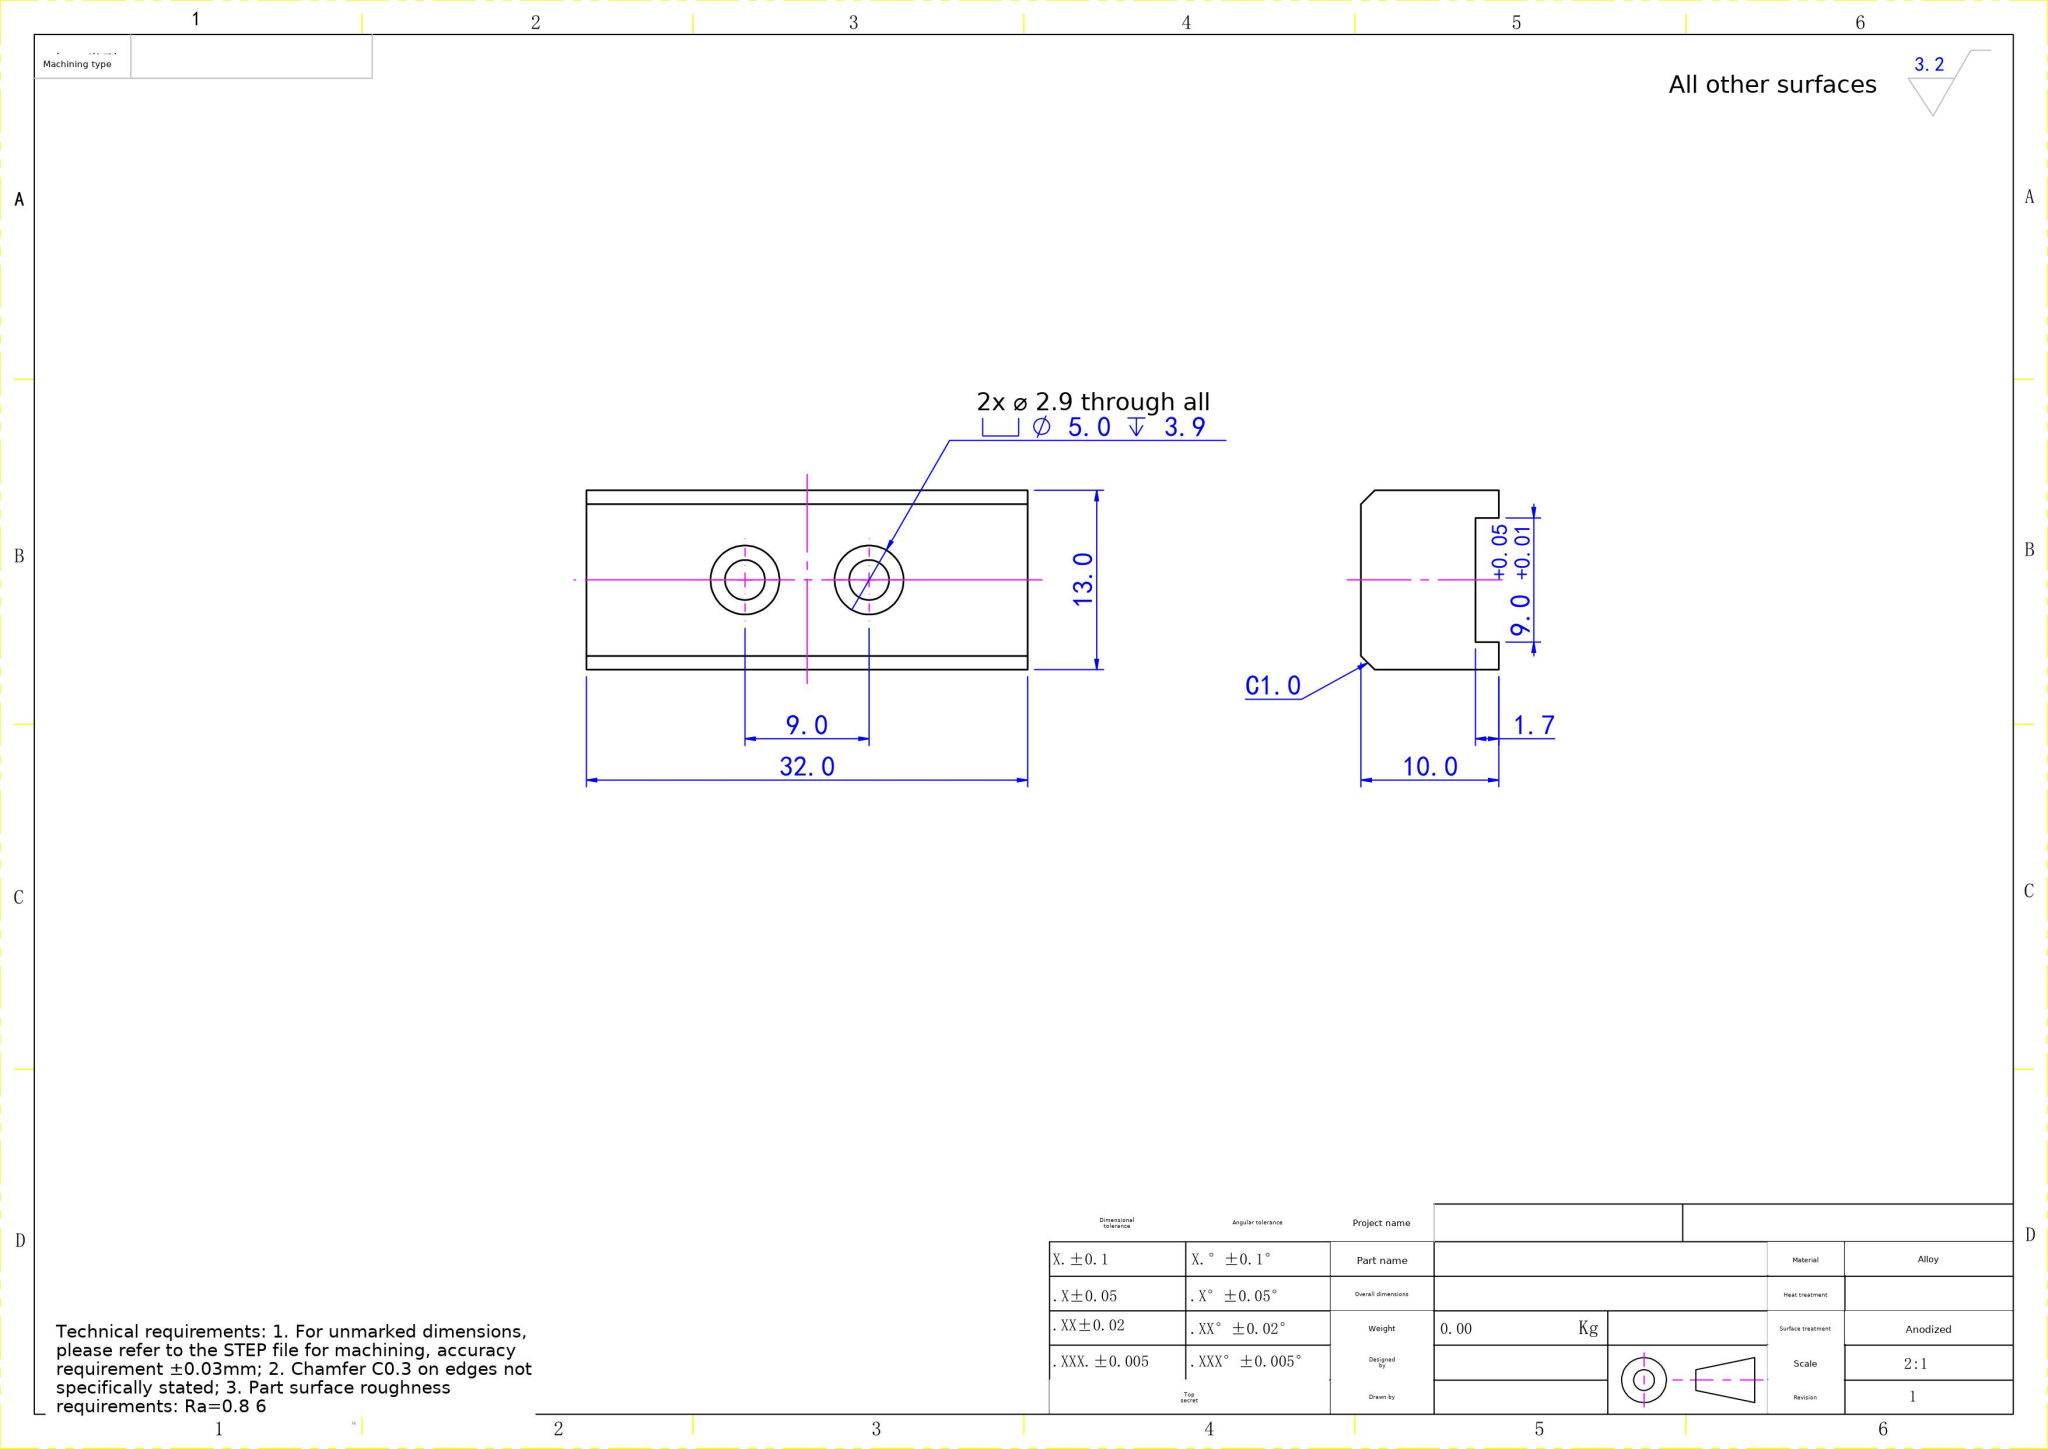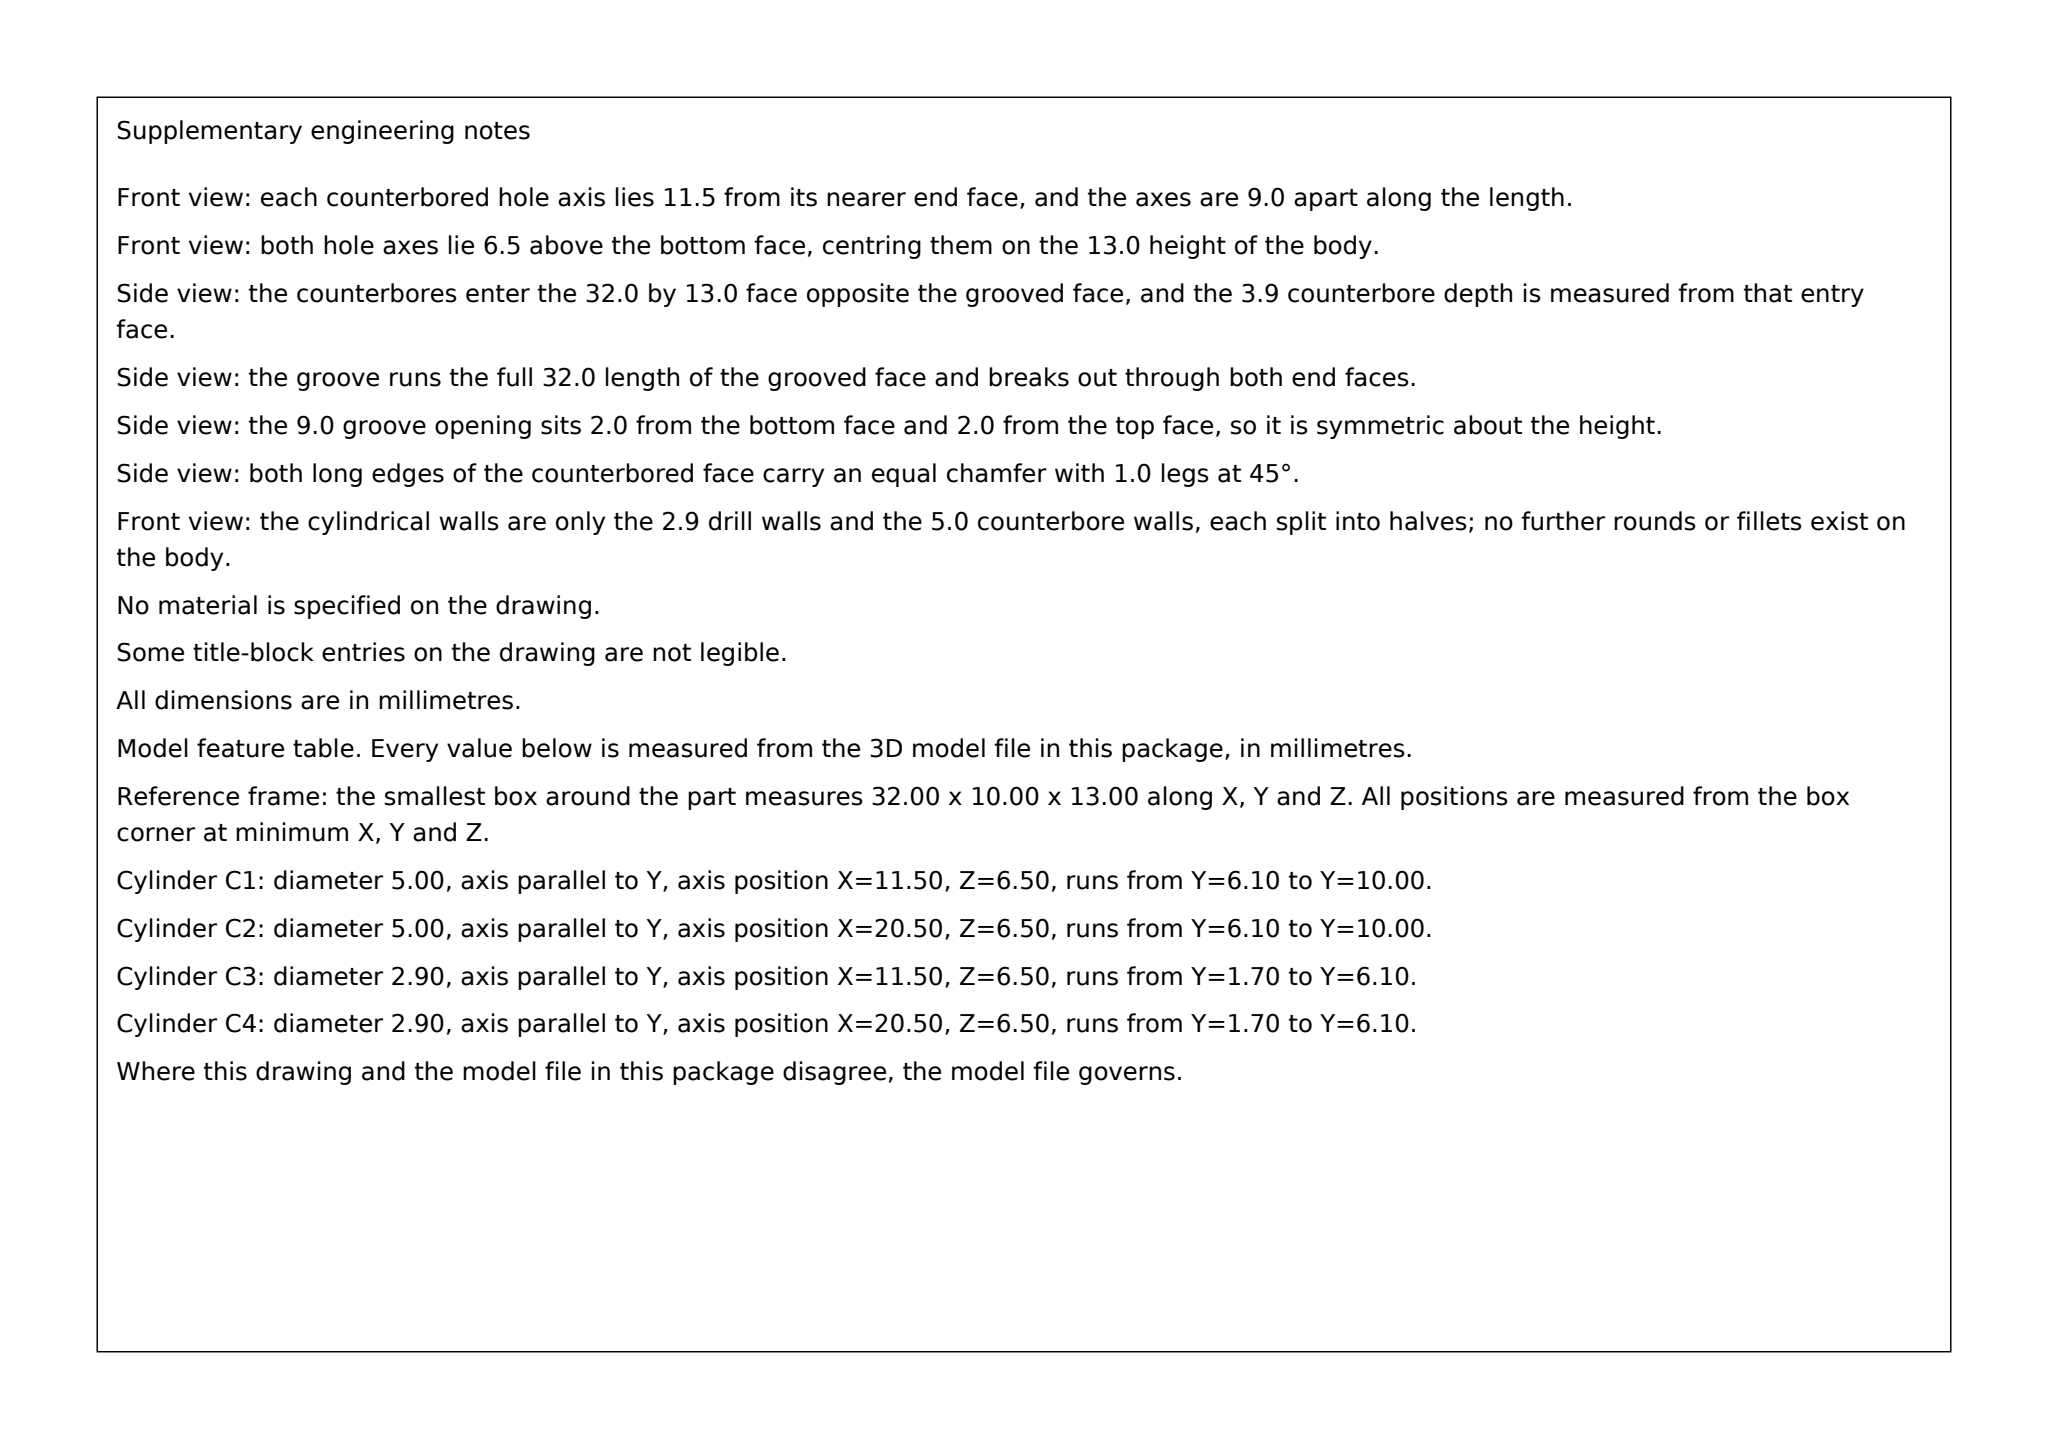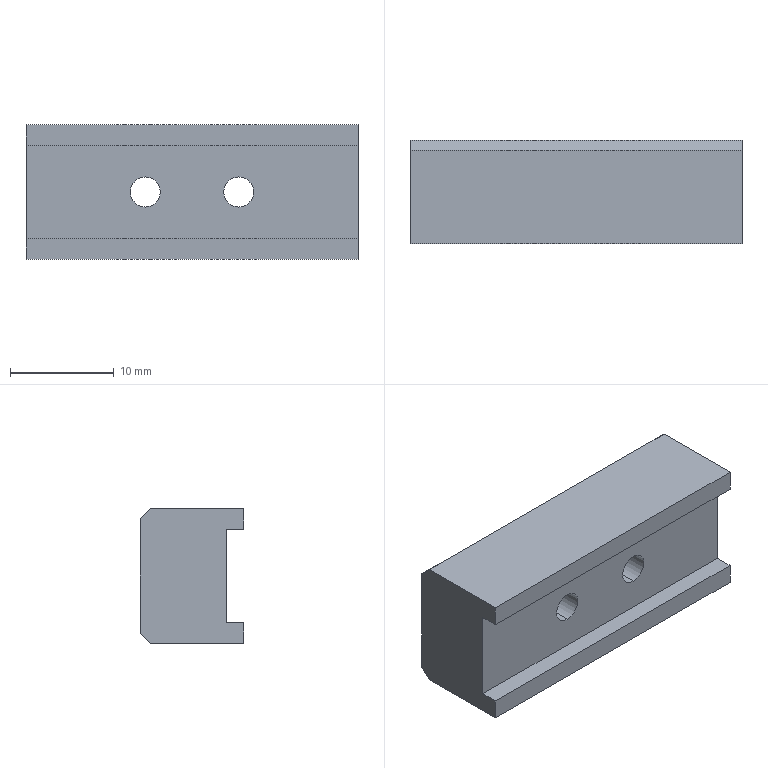Part | SolidWorks | mm | 1 solid | 22 faces | box 32 x 10 x 13 mm | volume 3427 mm3 | plane 14 | cylinder 8 | commonest cylinder face diameters 5 x4 2.9 x4
Drawing notes:
2X C'BORE Ø5.0 DP 3.9 FROM FACE OPP 1.7 STEP IN SIDE VIEW | from the solid: Ø5.0 y-axis cyl len 3.9 with floor plane y=6.1 (=10.0-3.9); Ø2.9 len 4.4 runs y=1.7 to 6.1, breaking out at the y=1.7 step face; bbox y=10.0
build123d program:
from build123d import *

# Parameters (mm, degrees)
SKETCH1_W                                         = 32
SKETCH1_H                                         = 10
BOSS_EXTRUDE1_DEPTH                               = 13
CUT_EXTRUDE1_DEPTH                                = 117.619
CUT_EXTRUDE1_DEPTH_BACK                           = 117.619
SKETCH2_W                                         = 9
SKETCH2_H                                         = 3.4
M2_5_HEX_SOCKET_HEAD_CAP_SCREW_CBORE1_D           = 2.9
M2_5_HEX_SOCKET_HEAD_CAP_SCREW_CBORE1_DEPTH       = 10
M2_5_HEX_SOCKET_HEAD_CAP_SCREW_CBORE1_CBORE_D     = 5
M2_5_HEX_SOCKET_HEAD_CAP_SCREW_CBORE1_CBORE_DEPTH = 3.9
CHAMFER1_SIZE                                     = 1


with BuildPart() as part:
    # Sketch1 → Boss-Extrude1 (new body)
    with BuildSketch(Plane.XY):
        with Locations((-5.72, -106.387)):
            Rectangle(SKETCH1_W, SKETCH1_H)
    extrude(amount=BOSS_EXTRUDE1_DEPTH)

    # Sketch2 → Cut-Extrude1 (cut, two sides: drawn at the far end of the back side and taken through both)
    with BuildSketch(Plane.ZY.offset(21.72).offset(-CUT_EXTRUDE1_DEPTH_BACK)):
        with Locations((6.5, -111.387)):
            Rectangle(SKETCH2_W, SKETCH2_H)
    extrude(amount=CUT_EXTRUDE1_DEPTH + CUT_EXTRUDE1_DEPTH_BACK, mode=Mode.SUBTRACT)

    # M2.5 Hex Socket Head Cap Screw CBORE1
    with Locations(Plane(origin=(0, -101.387, 0), x_dir=(1, 0, 0), z_dir=(0, 1, 0))):
        with Locations((-10.22, -6.5), (-1.22, -6.5)):
            CounterBoreHole(M2_5_HEX_SOCKET_HEAD_CAP_SCREW_CBORE1_D / 2, M2_5_HEX_SOCKET_HEAD_CAP_SCREW_CBORE1_CBORE_D / 2, M2_5_HEX_SOCKET_HEAD_CAP_SCREW_CBORE1_CBORE_DEPTH, depth=M2_5_HEX_SOCKET_HEAD_CAP_SCREW_CBORE1_DEPTH)

    # Chamfer1
    chamfer1_edges = [part.edges().sort_by_distance(p)[0] for p in [
        (-5.72, -101.387, 0),
        (-5.72, -101.387, 13),
    ]]
    chamfer(chamfer1_edges, length=CHAMFER1_SIZE)


solid = part.part